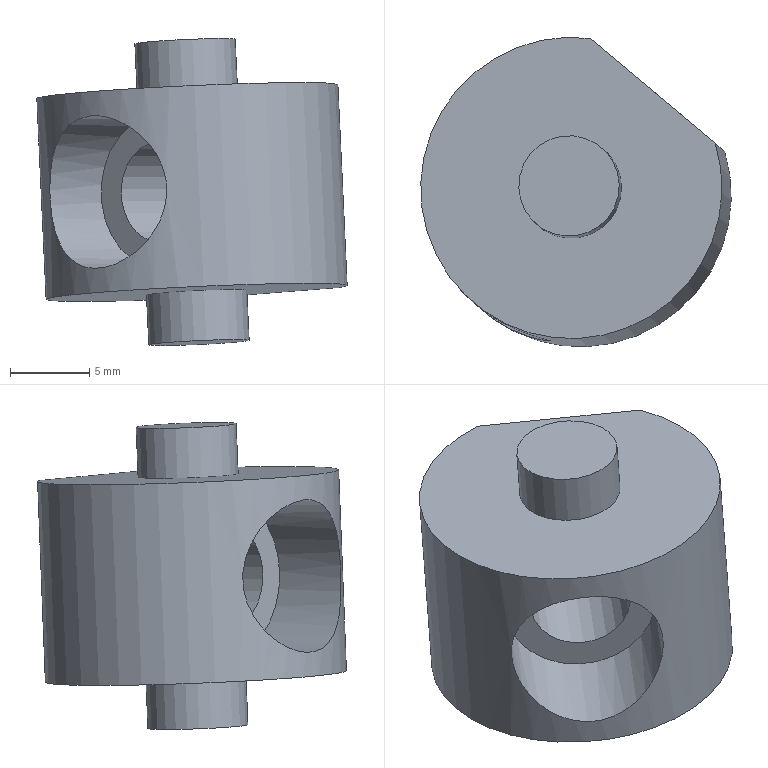Component | NX | ARTICULACION_B | 1 solid | 11 faces | box 19.62 x 19.53 x 19.4 mm | volume 2890 mm3 | plane 6 | cylinder 5 | commonest cylinder face diameters 6.35 x3 19.05 x1 9.652 x1
STEP:
#1=CARTESIAN_POINT('',(0.,0.,0.));
#2=DIRECTION('',(0.,0.,1.));
#3=DIRECTION('',(1.,0.,0.));
#4=AXIS2_PLACEMENT_3D('',#1,#2,#3);
#5=CARTESIAN_POINT('',(67.506,-0.9967,0.08803));
#6=VERTEX_POINT('',#5);
#7=CARTESIAN_POINT('',(75.41,-7.629,0.712));
#8=VERTEX_POINT('',#7);
#9=CARTESIAN_POINT('',(66.315,-10.442,0.4));
#10=DIRECTION('',(-0.04625,0.03881,0.9982));
#11=DIRECTION('',(0.7646,-0.6416,0.06037));
#12=AXIS2_PLACEMENT_3D('',#9,#10,#11);
#13=CIRCLE('',#12,9.525);
#14=CARTESIAN_POINT('',(65.728,-9.949,13.077));
#15=DIRECTION('',(0.04625,-0.03881,-0.9982));
#16=DIRECTION('',(-0.7646,0.6416,-0.06037));
#17=AXIS2_PLACEMENT_3D('',#14,#15,#16);
#18=CYLINDRICAL_SURFACE('',#17,9.525);
#19=CARTESIAN_POINT('',(9.425,12.7));
#20=DIRECTION('',(-1.,0.));
#21=VECTOR('',#20,1.);
#22=LINE('',#19,#21);
#23=(GEOMETRIC_REPRESENTATION_CONTEXT(2)PARAMETRIC_REPRESENTATION_CONTEXT()REPRESENTATION_CONTEXT('',''));
#24=DEFINITIONAL_REPRESENTATION('',(#22),#23);
#25=PCURVE('',#18,#24);
#26=CARTESIAN_POINT('',(66.315,-10.442,0.4));
#27=DIRECTION('',(-0.04625,0.03881,0.9982));
#28=DIRECTION('',(0.7646,-0.6416,0.06037));
#29=AXIS2_PLACEMENT_3D('',#26,#27,#28);
#30=PLANE('',#29);
#31=CARTESIAN_POINT('',(0.,0.));
#32=DIRECTION('',(1.,0.));
#33=AXIS2_PLACEMENT_2D('',#31,#32);
#34=CIRCLE('',#33,9.525);
#35=(GEOMETRIC_REPRESENTATION_CONTEXT(2)PARAMETRIC_REPRESENTATION_CONTEXT()REPRESENTATION_CONTEXT('',''));
#36=DEFINITIONAL_REPRESENTATION('',(#34),#35);
#37=PCURVE('',#30,#36);
#38=SURFACE_CURVE('',#13,(#25,#37),.PCURVE_S1.);
#39=EDGE_CURVE('',#6,#8,#38,.T.);
#40=ORIENTED_EDGE('',*,*,#39,.T.);
#41=CARTESIAN_POINT('',(74.822,-7.136,13.389));
#42=VERTEX_POINT('',#41);
#43=CARTESIAN_POINT('',(74.822,-7.136,13.389));
#44=DIRECTION('',(-0.04625,0.03881,0.9982));
#45=VECTOR('',#44,1.);
#46=LINE('',#43,#45);
#47=CARTESIAN_POINT('',(2.144,-0.));
#48=DIRECTION('',(0.,-1.));
#49=VECTOR('',#48,1.);
#50=LINE('',#47,#49);
#51=(GEOMETRIC_REPRESENTATION_CONTEXT(2)PARAMETRIC_REPRESENTATION_CONTEXT()REPRESENTATION_CONTEXT('',''));
#52=DEFINITIONAL_REPRESENTATION('',(#50),#51);
#53=PCURVE('',#18,#52);
#54=CARTESIAN_POINT('',(74.822,-7.136,13.389));
#55=DIRECTION('',(-0.6428,-0.766,0.));
#56=DIRECTION('',(0.04625,-0.03881,-0.9982));
#57=AXIS2_PLACEMENT_3D('',#54,#55,#56);
#58=PLANE('',#57);
#59=CARTESIAN_POINT('',(-0.,0.));
#60=DIRECTION('',(-1.,0.));
#61=VECTOR('',#60,1.);
#62=LINE('',#59,#61);
#63=(GEOMETRIC_REPRESENTATION_CONTEXT(2)PARAMETRIC_REPRESENTATION_CONTEXT()REPRESENTATION_CONTEXT('',''));
#64=DEFINITIONAL_REPRESENTATION('',(#62),#63);
#65=PCURVE('',#58,#64);
#66=SURFACE_CURVE('',#46,(#53,#65),.PCURVE_S1.);
#67=EDGE_CURVE('',#8,#42,#66,.T.);
#68=ORIENTED_EDGE('',*,*,#67,.T.);
#69=CARTESIAN_POINT('',(66.919,-0.5039,12.765));
#70=VERTEX_POINT('',#69);
#71=CARTESIAN_POINT('',(65.728,-9.949,13.077));
#72=DIRECTION('',(-0.04625,0.03881,0.9982));
#73=DIRECTION('',(0.7646,-0.6416,0.06037));
#74=AXIS2_PLACEMENT_3D('',#71,#72,#73);
#75=CIRCLE('',#74,9.525);
#76=CARTESIAN_POINT('',(9.425,0.));
#77=DIRECTION('',(-1.,-0.));
#78=VECTOR('',#77,1.);
#79=LINE('',#76,#78);
#80=(GEOMETRIC_REPRESENTATION_CONTEXT(2)PARAMETRIC_REPRESENTATION_CONTEXT()REPRESENTATION_CONTEXT('',''));
#81=DEFINITIONAL_REPRESENTATION('',(#79),#80);
#82=PCURVE('',#18,#81);
#83=CARTESIAN_POINT('',(65.728,-9.949,13.077));
#84=DIRECTION('',(-0.04625,0.03881,0.9982));
#85=DIRECTION('',(0.7646,-0.6416,0.06037));
#86=AXIS2_PLACEMENT_3D('',#83,#84,#85);
#87=PLANE('',#86);
#88=CARTESIAN_POINT('',(0.,0.));
#89=DIRECTION('',(1.,0.));
#90=AXIS2_PLACEMENT_2D('',#88,#89);
#91=CIRCLE('',#90,9.525);
#92=(GEOMETRIC_REPRESENTATION_CONTEXT(2)PARAMETRIC_REPRESENTATION_CONTEXT()REPRESENTATION_CONTEXT('',''));
#93=DEFINITIONAL_REPRESENTATION('',(#91),#92);
#94=PCURVE('',#87,#93);
#95=SURFACE_CURVE('',#75,(#82,#94),.PCURVE_S1.);
#96=EDGE_CURVE('',#70,#42,#95,.T.);
#97=ORIENTED_EDGE('',*,*,#96,.F.);
#98=CARTESIAN_POINT('',(66.919,-0.5039,12.765));
#99=DIRECTION('',(0.04625,-0.03881,-0.9982));
#100=VECTOR('',#99,1.);
#101=LINE('',#98,#100);
#102=CARTESIAN_POINT('',(7.28,0.));
#103=DIRECTION('',(0.,1.));
#104=VECTOR('',#103,1.);
#105=LINE('',#102,#104);
#106=(GEOMETRIC_REPRESENTATION_CONTEXT(2)PARAMETRIC_REPRESENTATION_CONTEXT()REPRESENTATION_CONTEXT('',''));
#107=DEFINITIONAL_REPRESENTATION('',(#105),#106);
#108=PCURVE('',#18,#107);
#109=CARTESIAN_POINT('',(0.,-10.336));
#110=DIRECTION('',(1.,-0.));
#111=VECTOR('',#110,1.);
#112=LINE('',#109,#111);
#113=(GEOMETRIC_REPRESENTATION_CONTEXT(2)PARAMETRIC_REPRESENTATION_CONTEXT()REPRESENTATION_CONTEXT('',''));
#114=DEFINITIONAL_REPRESENTATION('',(#112),#113);
#115=PCURVE('',#58,#114);
#116=SURFACE_CURVE('',#101,(#108,#115),.PCURVE_S1.);
#117=EDGE_CURVE('',#70,#6,#116,.T.);
#118=ORIENTED_EDGE('',*,*,#117,.T.);
#119=EDGE_LOOP('',(#40,#68,#97,#118));
#120=FACE_BOUND('',#119,.T.);
#121=CARTESIAN_POINT('',(59.676,-17.305,11.556));
#122=VERTEX_POINT('',#121);
#123=CARTESIAN_POINT('',(60.669,-18.138,11.634));
#124=CARTESIAN_POINT('',(58.683,-16.471,11.477));
#125=CARTESIAN_POINT('',(57.949,-15.468,10.863));
#126=CARTESIAN_POINT('',(57.125,-13.901,9.011));
#127=CARTESIAN_POINT('',(56.994,-13.343,7.741));
#128=CARTESIAN_POINT('',(57.11,-13.436,5.177));
#129=CARTESIAN_POINT('',(57.357,-14.092,3.956));
#130=CARTESIAN_POINT('',(58.341,-15.794,2.311));
#131=CARTESIAN_POINT('',(59.133,-16.847,1.847));
#132=CARTESIAN_POINT('',(61.09,-18.494,1.994));
#133=CARTESIAN_POINT('',(62.223,-19.057,2.608));
#134=CARTESIAN_POINT('',(63.917,-19.6,4.464));
#135=CARTESIAN_POINT('',(64.489,-19.632,5.741));
#136=CARTESIAN_POINT('',(64.378,-19.534,8.294));
#137=CARTESIAN_POINT('',(63.693,-19.406,9.518));
#138=CARTESIAN_POINT('',(61.833,-18.728,11.173));
#139=CARTESIAN_POINT('',(60.669,-18.138,11.634));
#140=CARTESIAN_POINT('',(58.683,-16.471,11.477));
#141=B_SPLINE_CURVE_WITH_KNOTS('',3,(#123,#124,#125,#126,#127,#128,#129,#130,#131,#132,#133,#134,#135,#136,#137,#138,#139,#140),.UNSPECIFIED.,.T.,.F.,(2,2,2,2,2,2,2,2,2,2,2),(-0.125,0.,0.125,0.25,0.375,0.5,0.625,0.75,0.875,1.,1.125),.UNSPECIFIED.);
#142=CARTESIAN_POINT('',(4.712,1.524));
#143=CARTESIAN_POINT('',(4.737,1.524));
#144=CARTESIAN_POINT('',(4.786,1.56));
#145=CARTESIAN_POINT('',(4.858,1.713));
#146=CARTESIAN_POINT('',(4.927,1.959));
#147=CARTESIAN_POINT('',(4.992,2.289));
#148=CARTESIAN_POINT('',(5.052,2.697));
#149=CARTESIAN_POINT('',(5.106,3.175));
#150=CARTESIAN_POINT('',(5.153,3.721));
#151=CARTESIAN_POINT('',(5.191,4.321));
#152=CARTESIAN_POINT('',(5.22,4.965));
#153=CARTESIAN_POINT('',(5.239,5.64));
#154=CARTESIAN_POINT('',(5.246,6.338));
#155=CARTESIAN_POINT('',(5.239,7.037));
#156=CARTESIAN_POINT('',(5.221,7.716));
#157=CARTESIAN_POINT('',(5.192,8.365));
#158=CARTESIAN_POINT('',(5.153,8.969));
#159=CARTESIAN_POINT('',(5.107,9.518));
#160=CARTESIAN_POINT('',(5.053,9.997));
#161=CARTESIAN_POINT('',(4.993,10.406));
#162=CARTESIAN_POINT('',(4.928,10.737));
#163=CARTESIAN_POINT('',(4.859,10.984));
#164=CARTESIAN_POINT('',(4.787,11.138));
#165=CARTESIAN_POINT('',(4.714,11.194));
#166=CARTESIAN_POINT('',(4.641,11.142));
#167=CARTESIAN_POINT('',(4.569,10.99));
#168=CARTESIAN_POINT('',(4.499,10.746));
#169=CARTESIAN_POINT('',(4.434,10.416));
#170=CARTESIAN_POINT('',(4.373,10.007));
#171=CARTESIAN_POINT('',(4.319,9.528));
#172=CARTESIAN_POINT('',(4.272,8.981));
#173=CARTESIAN_POINT('',(4.234,8.379));
#174=CARTESIAN_POINT('',(4.204,7.734));
#175=CARTESIAN_POINT('',(4.186,7.058));
#176=CARTESIAN_POINT('',(4.179,6.363));
#177=CARTESIAN_POINT('',(4.185,5.666));
#178=CARTESIAN_POINT('',(4.204,4.988));
#179=CARTESIAN_POINT('',(4.233,4.339));
#180=CARTESIAN_POINT('',(4.271,3.733));
#181=CARTESIAN_POINT('',(4.318,3.181));
#182=CARTESIAN_POINT('',(4.372,2.699));
#183=CARTESIAN_POINT('',(4.432,2.289));
#184=CARTESIAN_POINT('',(4.497,1.958));
#185=CARTESIAN_POINT('',(4.567,1.712));
#186=CARTESIAN_POINT('',(4.638,1.56));
#187=CARTESIAN_POINT('',(4.688,1.524));
#188=CARTESIAN_POINT('',(4.712,1.524));
#189=B_SPLINE_CURVE_WITH_KNOTS('',3,(#142,#143,#144,#145,#146,#147,#148,#149,#150,#151,#152,#153,#154,#155,#156,#157,#158,#159,#160,#161,#162,#163,#164,#165,#166,#167,#168,#169,#170,#171,#172,#173,#174,#175,#176,#177,#178,#179,#180,#181,#182,#183,#184,#185,#186,#187,#188),.UNSPECIFIED.,.T.,.F.,(4,1,1,1,1,1,1,1,1,1,1,1,1,1,1,1,1,1,1,1,1,1,1,1,1,1,1,1,1,1,1,1,1,1,1,1,1,1,1,1,1,1,1,1,4),(0.,0.02273,0.04545,0.06818,0.09091,0.1136,0.1364,0.1591,0.1818,0.2045,0.2273,0.25,0.2727,0.2955,0.3182,0.3409,0.3636,0.3864,0.4091,0.4318,0.4545,0.4773,0.5,0.5227,0.5455,0.5682,0.5909,0.6136,0.6364,0.6591,0.6818,0.7045,0.7273,0.75,0.7727,0.7955,0.8182,0.8409,0.8636,0.8864,0.9091,0.9318,0.9545,0.9773,1.),.QUASI_UNIFORM_KNOTS.);
#190=(GEOMETRIC_REPRESENTATION_CONTEXT(2)PARAMETRIC_REPRESENTATION_CONTEXT()REPRESENTATION_CONTEXT('',''));
#191=DEFINITIONAL_REPRESENTATION('',(#189),#190);
#192=PCURVE('',#18,#191);
#193=CARTESIAN_POINT('',(58.674,-18.951,6.738));
#194=DIRECTION('',(0.6428,0.766,0.));
#195=DIRECTION('',(-0.04625,0.03881,0.9982));
#196=AXIS2_PLACEMENT_3D('',#193,#194,#195);
#197=CYLINDRICAL_SURFACE('',#196,4.826);
#198=CARTESIAN_POINT('',(6.283,1.905));
#199=CARTESIAN_POINT('',(6.234,1.905));
#200=CARTESIAN_POINT('',(6.137,1.925));
#201=CARTESIAN_POINT('',(5.993,2.004));
#202=CARTESIAN_POINT('',(5.85,2.123));
#203=CARTESIAN_POINT('',(5.708,2.274));
#204=CARTESIAN_POINT('',(5.567,2.445));
#205=CARTESIAN_POINT('',(5.428,2.63));
#206=CARTESIAN_POINT('',(5.287,2.81));
#207=CARTESIAN_POINT('',(5.145,2.972));
#208=CARTESIAN_POINT('',(5.003,3.105));
#209=CARTESIAN_POINT('',(4.859,3.195));
#210=CARTESIAN_POINT('',(4.715,3.229));
#211=CARTESIAN_POINT('',(4.57,3.196));
#212=CARTESIAN_POINT('',(4.426,3.107));
#213=CARTESIAN_POINT('',(4.283,2.975));
#214=CARTESIAN_POINT('',(4.14,2.812));
#215=CARTESIAN_POINT('',(3.999,2.633));
#216=CARTESIAN_POINT('',(3.859,2.448));
#217=CARTESIAN_POINT('',(3.718,2.276));
#218=CARTESIAN_POINT('',(3.576,2.125));
#219=CARTESIAN_POINT('',(3.433,2.005));
#220=CARTESIAN_POINT('',(3.289,1.926));
#221=CARTESIAN_POINT('',(3.145,1.895));
#222=CARTESIAN_POINT('',(3.,1.924));
#223=CARTESIAN_POINT('',(2.856,2.002));
#224=CARTESIAN_POINT('',(2.712,2.121));
#225=CARTESIAN_POINT('',(2.569,2.272));
#226=CARTESIAN_POINT('',(2.427,2.444));
#227=CARTESIAN_POINT('',(2.287,2.629));
#228=CARTESIAN_POINT('',(2.146,2.809));
#229=CARTESIAN_POINT('',(2.004,2.972));
#230=CARTESIAN_POINT('',(1.861,3.104));
#231=CARTESIAN_POINT('',(1.718,3.194));
#232=CARTESIAN_POINT('',(1.573,3.229));
#233=CARTESIAN_POINT('',(1.429,3.196));
#234=CARTESIAN_POINT('',(1.285,3.108));
#235=CARTESIAN_POINT('',(1.142,2.976));
#236=CARTESIAN_POINT('',(0.9992,2.813));
#237=CARTESIAN_POINT('',(0.8574,2.632));
#238=CARTESIAN_POINT('',(0.7168,2.446));
#239=CARTESIAN_POINT('',(0.5754,2.274));
#240=CARTESIAN_POINT('',(0.4332,2.123));
#241=CARTESIAN_POINT('',(0.2901,2.004));
#242=CARTESIAN_POINT('',(0.146,1.925));
#243=CARTESIAN_POINT('',(0.04889,1.905));
#244=CARTESIAN_POINT('',(-0.,1.905));
#245=B_SPLINE_CURVE_WITH_KNOTS('',3,(#198,#199,#200,#201,#202,#203,#204,#205,#206,#207,#208,#209,#210,#211,#212,#213,#214,#215,#216,#217,#218,#219,#220,#221,#222,#223,#224,#225,#226,#227,#228,#229,#230,#231,#232,#233,#234,#235,#236,#237,#238,#239,#240,#241,#242,#243,#244),.UNSPECIFIED.,.F.,.F.,(4,1,1,1,1,1,1,1,1,1,1,1,1,1,1,1,1,1,1,1,1,1,1,1,1,1,1,1,1,1,1,1,1,1,1,1,1,1,1,1,1,1,1,1,4),(0.,0.02273,0.04545,0.06818,0.09091,0.1136,0.1364,0.1591,0.1818,0.2045,0.2273,0.25,0.2727,0.2955,0.3182,0.3409,0.3636,0.3864,0.4091,0.4318,0.4545,0.4773,0.5,0.5227,0.5455,0.5682,0.5909,0.6136,0.6364,0.6591,0.6818,0.7045,0.7273,0.75,0.7727,0.7955,0.8182,0.8409,0.8636,0.8864,0.9091,0.9318,0.9545,0.9773,1.),.QUASI_UNIFORM_KNOTS.);
#246=(GEOMETRIC_REPRESENTATION_CONTEXT(2)PARAMETRIC_REPRESENTATION_CONTEXT()REPRESENTATION_CONTEXT('',''));
#247=DEFINITIONAL_REPRESENTATION('',(#245),#246);
#248=PCURVE('',#197,#247);
#249=SURFACE_CURVE('',#141,(#192,#248),.PCURVE_S1.);
#250=EDGE_CURVE('',#122,#122,#249,.T.);
#251=ORIENTED_EDGE('',*,*,#250,.F.);
#252=EDGE_LOOP('',(#251));
#253=FACE_BOUND('',#252,.T.);
#254=ADVANCED_FACE('',(#120,#253),#18,.T.);
#255=CARTESIAN_POINT('',(71.311,-4.189,3.569));
#256=VERTEX_POINT('',#255);
#257=CARTESIAN_POINT('',(71.164,-4.066,6.738));
#258=DIRECTION('',(0.6428,0.766,-0.));
#259=DIRECTION('',(0.04625,-0.03881,-0.9982));
#260=AXIS2_PLACEMENT_3D('',#257,#258,#259);
#261=CIRCLE('',#260,3.175);
#262=CARTESIAN_POINT('',(55.817,-22.356,6.738));
#263=DIRECTION('',(0.6428,0.766,0.));
#264=DIRECTION('',(-0.04625,0.03881,0.9982));
#265=AXIS2_PLACEMENT_3D('',#262,#263,#264);
#266=CYLINDRICAL_SURFACE('',#265,3.175);
#267=CARTESIAN_POINT('',(3.142,23.876));
#268=DIRECTION('',(1.,0.));
#269=VECTOR('',#268,1.);
#270=LINE('',#267,#269);
#271=(GEOMETRIC_REPRESENTATION_CONTEXT(2)PARAMETRIC_REPRESENTATION_CONTEXT()REPRESENTATION_CONTEXT('',''));
#272=DEFINITIONAL_REPRESENTATION('',(#270),#271);
#273=PCURVE('',#266,#272);
#274=CARTESIAN_POINT('',(9.525,-5.168));
#275=CARTESIAN_POINT('',(9.525,-10.667));
#276=CARTESIAN_POINT('',(4.763,-7.918));
#277=CARTESIAN_POINT('',(-0.,-5.168));
#278=CARTESIAN_POINT('',(4.763,-2.419));
#279=CARTESIAN_POINT('',(9.525,0.3311));
#280=CARTESIAN_POINT('',(9.525,-5.168));
#281=(BOUNDED_CURVE()B_SPLINE_CURVE(2,(#274,#275,#276,#277,#278,#279,#280),.UNSPECIFIED.,.T.,.F.)B_SPLINE_CURVE_WITH_KNOTS((1,2,2,2,2,1),(-2.094,0.,2.094,4.189,6.283,8.378),.UNSPECIFIED.)CURVE()GEOMETRIC_REPRESENTATION_ITEM()RATIONAL_B_SPLINE_CURVE((1.,0.5,1.,0.5,1.,0.5,1.))REPRESENTATION_ITEM(''));
#282=(GEOMETRIC_REPRESENTATION_CONTEXT(2)PARAMETRIC_REPRESENTATION_CONTEXT()REPRESENTATION_CONTEXT('',''));
#283=DEFINITIONAL_REPRESENTATION('',(#281),#282);
#284=PCURVE('',#58,#283);
#285=SURFACE_CURVE('',#261,(#273,#284),.PCURVE_S1.);
#286=EDGE_CURVE('',#256,#256,#285,.T.);
#287=ORIENTED_EDGE('',*,*,#286,.F.);
#288=CARTESIAN_POINT('',(64.127,-12.751,3.569));
#289=VERTEX_POINT('',#288);
#290=CARTESIAN_POINT('',(64.127,-12.751,3.569));
#291=CARTESIAN_POINT('',(71.311,-4.189,3.569));
#292=B_SPLINE_CURVE_WITH_KNOTS('',1,(#290,#291),.UNSPECIFIED.,.F.,.F.,(2,2),(12.7,23.876),.PIECEWISE_BEZIER_KNOTS.);
#293=CARTESIAN_POINT('',(3.142,0.));
#294=DIRECTION('',(0.,1.));
#295=VECTOR('',#294,1.);
#296=LINE('',#293,#295);
#297=(GEOMETRIC_REPRESENTATION_CONTEXT(2)PARAMETRIC_REPRESENTATION_CONTEXT()REPRESENTATION_CONTEXT('',''));
#298=DEFINITIONAL_REPRESENTATION('',(#296),#297);
#299=PCURVE('',#266,#298);
#300=CARTESIAN_POINT('',(9.425,0.));
#301=DIRECTION('',(0.,1.));
#302=VECTOR('',#301,1.);
#303=LINE('',#300,#302);
#304=(GEOMETRIC_REPRESENTATION_CONTEXT(2)PARAMETRIC_REPRESENTATION_CONTEXT()REPRESENTATION_CONTEXT('',''));
#305=DEFINITIONAL_REPRESENTATION('',(#303),#304);
#306=PCURVE('',#266,#305);
#307=SEAM_CURVE('',#292,(#299,#306),.PCURVE_S1.);
#308=EDGE_CURVE('',#289,#256,#307,.T.);
#309=ORIENTED_EDGE('',*,*,#308,.F.);
#310=CARTESIAN_POINT('',(63.981,-12.628,6.738));
#311=DIRECTION('',(-0.6428,-0.766,0.));
#312=DIRECTION('',(0.04625,-0.03881,-0.9982));
#313=AXIS2_PLACEMENT_3D('',#310,#311,#312);
#314=CIRCLE('',#313,3.175);
#315=CARTESIAN_POINT('',(9.425,12.7));
#316=DIRECTION('',(-1.,0.));
#317=VECTOR('',#316,1.);
#318=LINE('',#315,#317);
#319=(GEOMETRIC_REPRESENTATION_CONTEXT(2)PARAMETRIC_REPRESENTATION_CONTEXT()REPRESENTATION_CONTEXT('',''));
#320=DEFINITIONAL_REPRESENTATION('',(#318),#319);
#321=PCURVE('',#266,#320);
#322=CARTESIAN_POINT('',(63.981,-12.628,6.738));
#323=DIRECTION('',(-0.6428,-0.766,0.));
#324=DIRECTION('',(0.04625,-0.03881,-0.9982));
#325=AXIS2_PLACEMENT_3D('',#322,#323,#324);
#326=PLANE('',#325);
#327=CARTESIAN_POINT('',(0.,0.));
#328=DIRECTION('',(1.,-0.));
#329=AXIS2_PLACEMENT_2D('',#327,#328);
#330=CIRCLE('',#329,3.175);
#331=(GEOMETRIC_REPRESENTATION_CONTEXT(2)PARAMETRIC_REPRESENTATION_CONTEXT()REPRESENTATION_CONTEXT('',''));
#332=DEFINITIONAL_REPRESENTATION('',(#330),#331);
#333=PCURVE('',#326,#332);
#334=SURFACE_CURVE('',#314,(#321,#333),.PCURVE_S1.);
#335=EDGE_CURVE('',#289,#289,#334,.T.);
#336=ORIENTED_EDGE('',*,*,#335,.F.);
#337=ORIENTED_EDGE('',*,*,#308,.T.);
#338=EDGE_LOOP('',(#287,#309,#336,#337));
#339=FACE_BOUND('',#338,.F.);
#340=ADVANCED_FACE('',(#339),#266,.F.);
#341=CARTESIAN_POINT('',(75.41,-7.629,0.712));
#342=DIRECTION('',(-0.7646,0.6416,-0.06037));
#343=VECTOR('',#342,1.);
#344=LINE('',#341,#343);
#345=CARTESIAN_POINT('',(12.7,0.));
#346=DIRECTION('',(0.,-1.));
#347=VECTOR('',#346,1.);
#348=LINE('',#345,#347);
#349=(GEOMETRIC_REPRESENTATION_CONTEXT(2)PARAMETRIC_REPRESENTATION_CONTEXT()REPRESENTATION_CONTEXT('',''));
#350=DEFINITIONAL_REPRESENTATION('',(#348),#349);
#351=PCURVE('',#58,#350);
#352=CARTESIAN_POINT('',(5.168,8.001));
#353=DIRECTION('',(-1.,-0.));
#354=VECTOR('',#353,1.);
#355=LINE('',#352,#354);
#356=(GEOMETRIC_REPRESENTATION_CONTEXT(2)PARAMETRIC_REPRESENTATION_CONTEXT()REPRESENTATION_CONTEXT('',''));
#357=DEFINITIONAL_REPRESENTATION('',(#355),#356);
#358=PCURVE('',#30,#357);
#359=SURFACE_CURVE('',#344,(#351,#358),.PCURVE_S1.);
#360=EDGE_CURVE('',#8,#6,#359,.T.);
#361=ORIENTED_EDGE('',*,*,#360,.T.);
#362=ORIENTED_EDGE('',*,*,#117,.F.);
#363=CARTESIAN_POINT('',(70.871,-3.82,13.077));
#364=DIRECTION('',(-0.7646,0.6416,-0.06037));
#365=VECTOR('',#364,1.);
#366=LINE('',#363,#365);
#367=CARTESIAN_POINT('',(-0.,-5.168));
#368=DIRECTION('',(0.,-1.));
#369=VECTOR('',#368,1.);
#370=LINE('',#367,#369);
#371=(GEOMETRIC_REPRESENTATION_CONTEXT(2)PARAMETRIC_REPRESENTATION_CONTEXT()REPRESENTATION_CONTEXT('',''));
#372=DEFINITIONAL_REPRESENTATION('',(#370),#371);
#373=PCURVE('',#58,#372);
#374=CARTESIAN_POINT('',(0.,8.001));
#375=DIRECTION('',(-1.,0.));
#376=VECTOR('',#375,1.);
#377=LINE('',#374,#376);
#378=(GEOMETRIC_REPRESENTATION_CONTEXT(2)PARAMETRIC_REPRESENTATION_CONTEXT()REPRESENTATION_CONTEXT('',''));
#379=DEFINITIONAL_REPRESENTATION('',(#377),#378);
#380=PCURVE('',#87,#379);
#381=SURFACE_CURVE('',#366,(#373,#380),.PCURVE_S1.);
#382=EDGE_CURVE('',#42,#70,#381,.T.);
#383=ORIENTED_EDGE('',*,*,#382,.F.);
#384=ORIENTED_EDGE('',*,*,#67,.F.);
#385=EDGE_LOOP('',(#361,#362,#383,#384));
#386=FACE_BOUND('',#385,.T.);
#387=ORIENTED_EDGE('',*,*,#286,.F.);
#388=EDGE_LOOP('',(#387));
#389=FACE_BOUND('',#388,.T.);
#390=ADVANCED_FACE('',(#386,#389),#58,.F.);
#391=ORIENTED_EDGE('',*,*,#382,.T.);
#392=ORIENTED_EDGE('',*,*,#96,.T.);
#393=EDGE_LOOP('',(#391,#392));
#394=FACE_BOUND('',#393,.T.);
#395=CARTESIAN_POINT('',(68.155,-11.986,13.269));
#396=VERTEX_POINT('',#395);
#397=CARTESIAN_POINT('',(65.728,-9.949,13.077));
#398=DIRECTION('',(0.04625,-0.03881,-0.9982));
#399=DIRECTION('',(0.7646,-0.6416,0.06037));
#400=AXIS2_PLACEMENT_3D('',#397,#398,#399);
#401=CIRCLE('',#400,3.175);
#402=CARTESIAN_POINT('',(3.175,0.));
#403=CARTESIAN_POINT('',(3.175,-5.499));
#404=CARTESIAN_POINT('',(-1.587,-2.75));
#405=CARTESIAN_POINT('',(-6.35,-0.));
#406=CARTESIAN_POINT('',(-1.587,2.75));
#407=CARTESIAN_POINT('',(3.175,5.499));
#408=CARTESIAN_POINT('',(3.175,0.));
#409=(BOUNDED_CURVE()B_SPLINE_CURVE(2,(#402,#403,#404,#405,#406,#407,#408),.UNSPECIFIED.,.T.,.F.)B_SPLINE_CURVE_WITH_KNOTS((1,2,2,2,2,1),(-2.094,0.,2.094,4.189,6.283,8.378),.UNSPECIFIED.)CURVE()GEOMETRIC_REPRESENTATION_ITEM()RATIONAL_B_SPLINE_CURVE((1.,0.5,1.,0.5,1.,0.5,1.))REPRESENTATION_ITEM(''));
#410=(GEOMETRIC_REPRESENTATION_CONTEXT(2)PARAMETRIC_REPRESENTATION_CONTEXT()REPRESENTATION_CONTEXT('',''));
#411=DEFINITIONAL_REPRESENTATION('',(#409),#410);
#412=PCURVE('',#87,#411);
#413=CARTESIAN_POINT('',(65.581,-9.826,16.246));
#414=DIRECTION('',(0.04625,-0.03881,-0.9982));
#415=DIRECTION('',(-0.7646,0.6416,-0.06037));
#416=AXIS2_PLACEMENT_3D('',#413,#414,#415);
#417=CYLINDRICAL_SURFACE('',#416,3.175);
#418=CARTESIAN_POINT('',(3.142,3.175));
#419=DIRECTION('',(1.,0.));
#420=VECTOR('',#419,1.);
#421=LINE('',#418,#420);
#422=(GEOMETRIC_REPRESENTATION_CONTEXT(2)PARAMETRIC_REPRESENTATION_CONTEXT()REPRESENTATION_CONTEXT('',''));
#423=DEFINITIONAL_REPRESENTATION('',(#421),#422);
#424=PCURVE('',#417,#423);
#425=SURFACE_CURVE('',#401,(#412,#424),.PCURVE_S1.);
#426=EDGE_CURVE('',#396,#396,#425,.T.);
#427=ORIENTED_EDGE('',*,*,#426,.T.);
#428=EDGE_LOOP('',(#427));
#429=FACE_BOUND('',#428,.T.);
#430=ADVANCED_FACE('',(#394,#429),#87,.T.);
#431=ORIENTED_EDGE('',*,*,#39,.F.);
#432=ORIENTED_EDGE('',*,*,#360,.F.);
#433=EDGE_LOOP('',(#431,#432));
#434=FACE_BOUND('',#433,.T.);
#435=CARTESIAN_POINT('',(68.743,-12.479,0.5917));
#436=VERTEX_POINT('',#435);
#437=CARTESIAN_POINT('',(66.315,-10.442,0.4));
#438=DIRECTION('',(0.04625,-0.03881,-0.9982));
#439=DIRECTION('',(0.7646,-0.6416,0.06037));
#440=AXIS2_PLACEMENT_3D('',#437,#438,#439);
#441=CIRCLE('',#440,3.175);
#442=CARTESIAN_POINT('',(3.175,0.));
#443=CARTESIAN_POINT('',(3.175,-5.499));
#444=CARTESIAN_POINT('',(-1.587,-2.75));
#445=CARTESIAN_POINT('',(-6.35,-0.));
#446=CARTESIAN_POINT('',(-1.587,2.75));
#447=CARTESIAN_POINT('',(3.175,5.499));
#448=CARTESIAN_POINT('',(3.175,0.));
#449=(BOUNDED_CURVE()B_SPLINE_CURVE(2,(#442,#443,#444,#445,#446,#447,#448),.UNSPECIFIED.,.T.,.F.)B_SPLINE_CURVE_WITH_KNOTS((1,2,2,2,2,1),(-2.094,0.,2.094,4.189,6.283,8.378),.UNSPECIFIED.)CURVE()GEOMETRIC_REPRESENTATION_ITEM()RATIONAL_B_SPLINE_CURVE((1.,0.5,1.,0.5,1.,0.5,1.))REPRESENTATION_ITEM(''));
#450=(GEOMETRIC_REPRESENTATION_CONTEXT(2)PARAMETRIC_REPRESENTATION_CONTEXT()REPRESENTATION_CONTEXT('',''));
#451=DEFINITIONAL_REPRESENTATION('',(#449),#450);
#452=PCURVE('',#30,#451);
#453=CARTESIAN_POINT('',(65.581,-9.826,16.246));
#454=DIRECTION('',(0.04625,-0.03881,-0.9982));
#455=DIRECTION('',(-0.7646,0.6416,-0.06037));
#456=AXIS2_PLACEMENT_3D('',#453,#454,#455);
#457=CYLINDRICAL_SURFACE('',#456,3.175);
#458=CARTESIAN_POINT('',(3.142,15.875));
#459=DIRECTION('',(1.,0.));
#460=VECTOR('',#459,1.);
#461=LINE('',#458,#460);
#462=(GEOMETRIC_REPRESENTATION_CONTEXT(2)PARAMETRIC_REPRESENTATION_CONTEXT()REPRESENTATION_CONTEXT('',''));
#463=DEFINITIONAL_REPRESENTATION('',(#461),#462);
#464=PCURVE('',#457,#463);
#465=SURFACE_CURVE('',#441,(#452,#464),.PCURVE_S1.);
#466=EDGE_CURVE('',#436,#436,#465,.T.);
#467=ORIENTED_EDGE('',*,*,#466,.F.);
#468=EDGE_LOOP('',(#467));
#469=FACE_BOUND('',#468,.T.);
#470=ADVANCED_FACE('',(#434,#469),#30,.F.);
#471=CARTESIAN_POINT('',(68.89,-12.602,-2.577));
#472=VERTEX_POINT('',#471);
#473=CARTESIAN_POINT('',(66.462,-10.565,-2.769));
#474=DIRECTION('',(-0.04625,0.03881,0.9982));
#475=DIRECTION('',(0.7646,-0.6416,0.06037));
#476=AXIS2_PLACEMENT_3D('',#473,#474,#475);
#477=CIRCLE('',#476,3.175);
#478=CARTESIAN_POINT('',(66.462,-10.565,-2.769));
#479=DIRECTION('',(-0.04625,0.03881,0.9982));
#480=DIRECTION('',(0.7646,-0.6416,0.06037));
#481=AXIS2_PLACEMENT_3D('',#478,#479,#480);
#482=PLANE('',#481);
#483=CARTESIAN_POINT('',(0.,0.));
#484=DIRECTION('',(1.,0.));
#485=AXIS2_PLACEMENT_2D('',#483,#484);
#486=CIRCLE('',#485,3.175);
#487=(GEOMETRIC_REPRESENTATION_CONTEXT(2)PARAMETRIC_REPRESENTATION_CONTEXT()REPRESENTATION_CONTEXT('',''));
#488=DEFINITIONAL_REPRESENTATION('',(#486),#487);
#489=PCURVE('',#482,#488);
#490=CARTESIAN_POINT('',(9.425,19.05));
#491=DIRECTION('',(-1.,0.));
#492=VECTOR('',#491,1.);
#493=LINE('',#490,#492);
#494=(GEOMETRIC_REPRESENTATION_CONTEXT(2)PARAMETRIC_REPRESENTATION_CONTEXT()REPRESENTATION_CONTEXT('',''));
#495=DEFINITIONAL_REPRESENTATION('',(#493),#494);
#496=PCURVE('',#457,#495);
#497=SURFACE_CURVE('',#477,(#489,#496),.PCURVE_S1.);
#498=EDGE_CURVE('',#472,#472,#497,.T.);
#499=ORIENTED_EDGE('',*,*,#498,.F.);
#500=EDGE_LOOP('',(#499));
#501=FACE_BOUND('',#500,.T.);
#502=ADVANCED_FACE('',(#501),#482,.F.);
#503=ORIENTED_EDGE('',*,*,#498,.T.);
#504=CARTESIAN_POINT('',(68.743,-12.479,0.5917));
#505=CARTESIAN_POINT('',(68.89,-12.602,-2.577));
#506=B_SPLINE_CURVE_WITH_KNOTS('',1,(#504,#505),.UNSPECIFIED.,.F.,.F.,(2,2),(15.875,19.05),.PIECEWISE_BEZIER_KNOTS.);
#507=CARTESIAN_POINT('',(3.142,0.));
#508=DIRECTION('',(0.,1.));
#509=VECTOR('',#508,1.);
#510=LINE('',#507,#509);
#511=(GEOMETRIC_REPRESENTATION_CONTEXT(2)PARAMETRIC_REPRESENTATION_CONTEXT()REPRESENTATION_CONTEXT('',''));
#512=DEFINITIONAL_REPRESENTATION('',(#510),#511);
#513=PCURVE('',#457,#512);
#514=CARTESIAN_POINT('',(9.425,0.));
#515=DIRECTION('',(0.,1.));
#516=VECTOR('',#515,1.);
#517=LINE('',#514,#516);
#518=(GEOMETRIC_REPRESENTATION_CONTEXT(2)PARAMETRIC_REPRESENTATION_CONTEXT()REPRESENTATION_CONTEXT('',''));
#519=DEFINITIONAL_REPRESENTATION('',(#517),#518);
#520=PCURVE('',#457,#519);
#521=SEAM_CURVE('',#506,(#513,#520),.PCURVE_S1.);
#522=EDGE_CURVE('',#436,#472,#521,.T.);
#523=ORIENTED_EDGE('',*,*,#522,.F.);
#524=ORIENTED_EDGE('',*,*,#466,.T.);
#525=ORIENTED_EDGE('',*,*,#522,.T.);
#526=EDGE_LOOP('',(#503,#523,#524,#525));
#527=FACE_BOUND('',#526,.T.);
#528=ADVANCED_FACE('',(#527),#457,.T.);
#529=ORIENTED_EDGE('',*,*,#426,.F.);
#530=CARTESIAN_POINT('',(68.009,-11.863,16.438));
#531=VERTEX_POINT('',#530);
#532=CARTESIAN_POINT('',(68.009,-11.863,16.438));
#533=CARTESIAN_POINT('',(68.155,-11.986,13.269));
#534=B_SPLINE_CURVE_WITH_KNOTS('',1,(#532,#533),.UNSPECIFIED.,.F.,.F.,(2,2),(0.,3.175),.PIECEWISE_BEZIER_KNOTS.);
#535=CARTESIAN_POINT('',(3.142,0.));
#536=DIRECTION('',(0.,1.));
#537=VECTOR('',#536,1.);
#538=LINE('',#535,#537);
#539=(GEOMETRIC_REPRESENTATION_CONTEXT(2)PARAMETRIC_REPRESENTATION_CONTEXT()REPRESENTATION_CONTEXT('',''));
#540=DEFINITIONAL_REPRESENTATION('',(#538),#539);
#541=PCURVE('',#417,#540);
#542=CARTESIAN_POINT('',(9.425,0.));
#543=DIRECTION('',(0.,1.));
#544=VECTOR('',#543,1.);
#545=LINE('',#542,#544);
#546=(GEOMETRIC_REPRESENTATION_CONTEXT(2)PARAMETRIC_REPRESENTATION_CONTEXT()REPRESENTATION_CONTEXT('',''));
#547=DEFINITIONAL_REPRESENTATION('',(#545),#546);
#548=PCURVE('',#417,#547);
#549=SEAM_CURVE('',#534,(#541,#548),.PCURVE_S1.);
#550=EDGE_CURVE('',#531,#396,#549,.T.);
#551=ORIENTED_EDGE('',*,*,#550,.F.);
#552=CARTESIAN_POINT('',(65.581,-9.826,16.246));
#553=DIRECTION('',(-0.04625,0.03881,0.9982));
#554=DIRECTION('',(0.7646,-0.6416,0.06037));
#555=AXIS2_PLACEMENT_3D('',#552,#553,#554);
#556=CIRCLE('',#555,3.175);
#557=CARTESIAN_POINT('',(9.425,0.));
#558=DIRECTION('',(-1.,0.));
#559=VECTOR('',#558,1.);
#560=LINE('',#557,#559);
#561=(GEOMETRIC_REPRESENTATION_CONTEXT(2)PARAMETRIC_REPRESENTATION_CONTEXT()REPRESENTATION_CONTEXT('',''));
#562=DEFINITIONAL_REPRESENTATION('',(#560),#561);
#563=PCURVE('',#417,#562);
#564=CARTESIAN_POINT('',(65.581,-9.826,16.246));
#565=DIRECTION('',(-0.04625,0.03881,0.9982));
#566=DIRECTION('',(0.7646,-0.6416,0.06037));
#567=AXIS2_PLACEMENT_3D('',#564,#565,#566);
#568=PLANE('',#567);
#569=CARTESIAN_POINT('',(0.,0.));
#570=DIRECTION('',(1.,0.));
#571=AXIS2_PLACEMENT_2D('',#569,#570);
#572=CIRCLE('',#571,3.175);
#573=(GEOMETRIC_REPRESENTATION_CONTEXT(2)PARAMETRIC_REPRESENTATION_CONTEXT()REPRESENTATION_CONTEXT('',''));
#574=DEFINITIONAL_REPRESENTATION('',(#572),#573);
#575=PCURVE('',#568,#574);
#576=SURFACE_CURVE('',#556,(#563,#575),.PCURVE_S1.);
#577=EDGE_CURVE('',#531,#531,#576,.T.);
#578=ORIENTED_EDGE('',*,*,#577,.F.);
#579=ORIENTED_EDGE('',*,*,#550,.T.);
#580=EDGE_LOOP('',(#529,#551,#578,#579));
#581=FACE_BOUND('',#580,.T.);
#582=ADVANCED_FACE('',(#581),#417,.T.);
#583=ORIENTED_EDGE('',*,*,#577,.T.);
#584=EDGE_LOOP('',(#583));
#585=FACE_BOUND('',#584,.T.);
#586=ADVANCED_FACE('',(#585),#568,.T.);
#587=CARTESIAN_POINT('',(63.757,-12.44,11.556));
#588=VERTEX_POINT('',#587);
#589=CARTESIAN_POINT('',(67.671,-15.724,7.03));
#590=VERTEX_POINT('',#589);
#591=CARTESIAN_POINT('',(63.981,-12.628,6.738));
#592=DIRECTION('',(0.6428,0.766,0.));
#593=DIRECTION('',(0.7646,-0.6416,0.06037));
#594=AXIS2_PLACEMENT_3D('',#591,#592,#593);
#595=CIRCLE('',#594,4.826);
#596=CARTESIAN_POINT('',(-4.712,8.255));
#597=DIRECTION('',(1.,0.));
#598=VECTOR('',#597,1.);
#599=LINE('',#596,#598);
#600=(GEOMETRIC_REPRESENTATION_CONTEXT(2)PARAMETRIC_REPRESENTATION_CONTEXT()REPRESENTATION_CONTEXT('',''));
#601=DEFINITIONAL_REPRESENTATION('',(#599),#600);
#602=PCURVE('',#197,#601);
#603=CARTESIAN_POINT('',(0.,4.826));
#604=CARTESIAN_POINT('',(8.359,4.826));
#605=CARTESIAN_POINT('',(4.179,-2.413));
#606=CARTESIAN_POINT('',(0.,-9.652));
#607=CARTESIAN_POINT('',(-4.179,-2.413));
#608=CARTESIAN_POINT('',(-8.359,4.826));
#609=CARTESIAN_POINT('',(0.,4.826));
#610=(BOUNDED_CURVE()B_SPLINE_CURVE(2,(#603,#604,#605,#606,#607,#608,#609),.UNSPECIFIED.,.T.,.F.)B_SPLINE_CURVE_WITH_KNOTS((1,2,2,2,2,1),(-2.094,0.,2.094,4.189,6.283,8.378),.UNSPECIFIED.)CURVE()GEOMETRIC_REPRESENTATION_ITEM()RATIONAL_B_SPLINE_CURVE((1.,0.5,1.,0.5,1.,0.5,1.))REPRESENTATION_ITEM(''));
#611=(GEOMETRIC_REPRESENTATION_CONTEXT(2)PARAMETRIC_REPRESENTATION_CONTEXT()REPRESENTATION_CONTEXT('',''));
#612=DEFINITIONAL_REPRESENTATION('',(#610),#611);
#613=PCURVE('',#326,#612);
#614=SURFACE_CURVE('',#595,(#602,#613),.PCURVE_S1.);
#615=EDGE_CURVE('',#588,#590,#614,.T.);
#616=ORIENTED_EDGE('',*,*,#615,.F.);
#617=CARTESIAN_POINT('',(59.676,-17.305,11.556));
#618=CARTESIAN_POINT('',(63.757,-12.44,11.556));
#619=B_SPLINE_CURVE_WITH_KNOTS('',1,(#617,#618),.UNSPECIFIED.,.F.,.F.,(2,2),(1.905,8.255),.PIECEWISE_BEZIER_KNOTS.);
#620=CARTESIAN_POINT('',(-0.,0.));
#621=DIRECTION('',(0.,1.));
#622=VECTOR('',#621,1.);
#623=LINE('',#620,#622);
#624=(GEOMETRIC_REPRESENTATION_CONTEXT(2)PARAMETRIC_REPRESENTATION_CONTEXT()REPRESENTATION_CONTEXT('',''));
#625=DEFINITIONAL_REPRESENTATION('',(#623),#624);
#626=PCURVE('',#197,#625);
#627=CARTESIAN_POINT('',(6.283,0.));
#628=DIRECTION('',(0.,1.));
#629=VECTOR('',#628,1.);
#630=LINE('',#627,#629);
#631=(GEOMETRIC_REPRESENTATION_CONTEXT(2)PARAMETRIC_REPRESENTATION_CONTEXT()REPRESENTATION_CONTEXT('',''));
#632=DEFINITIONAL_REPRESENTATION('',(#630),#631);
#633=PCURVE('',#197,#632);
#634=SEAM_CURVE('',#619,(#626,#633),.PCURVE_S1.);
#635=EDGE_CURVE('',#122,#588,#634,.T.);
#636=ORIENTED_EDGE('',*,*,#635,.F.);
#637=ORIENTED_EDGE('',*,*,#250,.F.);
#638=ORIENTED_EDGE('',*,*,#635,.T.);
#639=CARTESIAN_POINT('',(63.981,-12.628,6.738));
#640=DIRECTION('',(0.6428,0.766,0.));
#641=DIRECTION('',(0.7646,-0.6416,0.06037));
#642=AXIS2_PLACEMENT_3D('',#639,#640,#641);
#643=CIRCLE('',#642,4.826);
#644=CARTESIAN_POINT('',(1.571,8.255));
#645=DIRECTION('',(1.,0.));
#646=VECTOR('',#645,1.);
#647=LINE('',#644,#646);
#648=(GEOMETRIC_REPRESENTATION_CONTEXT(2)PARAMETRIC_REPRESENTATION_CONTEXT()REPRESENTATION_CONTEXT('',''));
#649=DEFINITIONAL_REPRESENTATION('',(#647),#648);
#650=PCURVE('',#197,#649);
#651=CARTESIAN_POINT('',(0.,4.826));
#652=CARTESIAN_POINT('',(8.359,4.826));
#653=CARTESIAN_POINT('',(4.179,-2.413));
#654=CARTESIAN_POINT('',(0.,-9.652));
#655=CARTESIAN_POINT('',(-4.179,-2.413));
#656=CARTESIAN_POINT('',(-8.359,4.826));
#657=CARTESIAN_POINT('',(0.,4.826));
#658=(BOUNDED_CURVE()B_SPLINE_CURVE(2,(#651,#652,#653,#654,#655,#656,#657),.UNSPECIFIED.,.T.,.F.)B_SPLINE_CURVE_WITH_KNOTS((1,2,2,2,2,1),(-2.094,0.,2.094,4.189,6.283,8.378),.UNSPECIFIED.)CURVE()GEOMETRIC_REPRESENTATION_ITEM()RATIONAL_B_SPLINE_CURVE((1.,0.5,1.,0.5,1.,0.5,1.))REPRESENTATION_ITEM(''));
#659=(GEOMETRIC_REPRESENTATION_CONTEXT(2)PARAMETRIC_REPRESENTATION_CONTEXT()REPRESENTATION_CONTEXT('',''));
#660=DEFINITIONAL_REPRESENTATION('',(#658),#659);
#661=PCURVE('',#326,#660);
#662=SURFACE_CURVE('',#643,(#650,#661),.PCURVE_S1.);
#663=EDGE_CURVE('',#590,#588,#662,.T.);
#664=ORIENTED_EDGE('',*,*,#663,.F.);
#665=EDGE_LOOP('',(#616,#636,#637,#638,#664));
#666=FACE_BOUND('',#665,.F.);
#667=ADVANCED_FACE('',(#666),#197,.F.);
#668=ORIENTED_EDGE('',*,*,#335,.F.);
#669=EDGE_LOOP('',(#668));
#670=FACE_BOUND('',#669,.T.);
#671=ORIENTED_EDGE('',*,*,#663,.F.);
#672=ORIENTED_EDGE('',*,*,#615,.F.);
#673=EDGE_LOOP('',(#671,#672));
#674=FACE_BOUND('',#673,.T.);
#675=ADVANCED_FACE('',(#670,#674),#326,.T.);
#676=CLOSED_SHELL('',(#254,#340,#390,#430,#470,#502,#528,#582,#586,#667,#675));
#677=MANIFOLD_SOLID_BREP('',#676);
#678=(LENGTH_UNIT()NAMED_UNIT(*)SI_UNIT(.MILLI.,.METRE.));
#679=UNCERTAINTY_MEASURE_WITH_UNIT(LENGTH_MEASURE(0.0005),#678,'','');
#680=(NAMED_UNIT(*)PLANE_ANGLE_UNIT()SI_UNIT($,.RADIAN.));
#681=(NAMED_UNIT(*)SI_UNIT($,.STERADIAN.)SOLID_ANGLE_UNIT());
#682=(GEOMETRIC_REPRESENTATION_CONTEXT(3)GLOBAL_UNCERTAINTY_ASSIGNED_CONTEXT((#679))GLOBAL_UNIT_ASSIGNED_CONTEXT((#678,#680,#681))REPRESENTATION_CONTEXT('',''));
#683=ADVANCED_BREP_SHAPE_REPRESENTATION('',(#4,#677),#682);